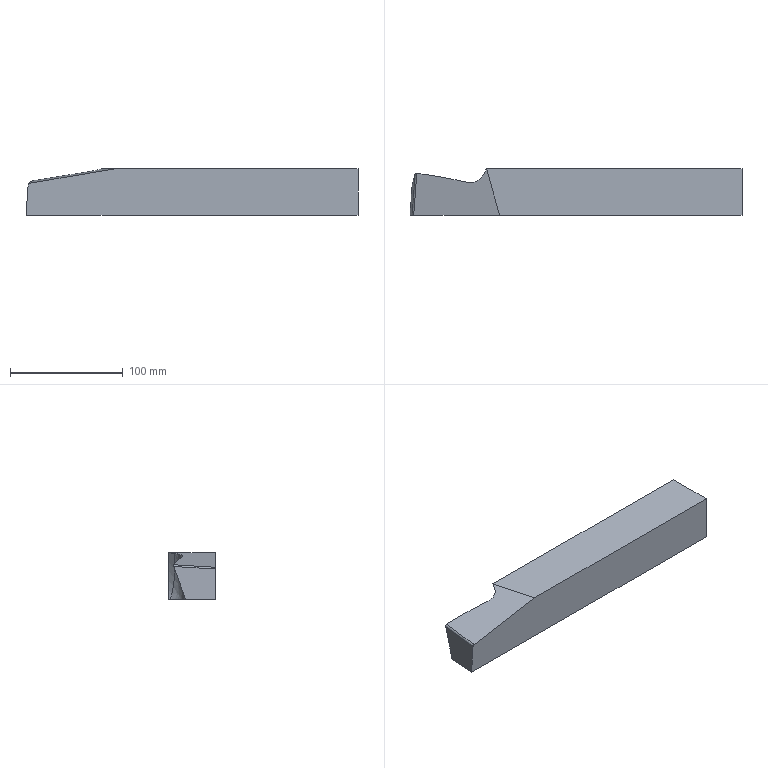Component | SolidWorks | LatheTool-1 | 1 solid | 11 faces | box 294.48 x 41.35 x 41.35 mm | volume 452255 mm3 | plane 7 | spline 3 | cylinder 1 | commonest cylinder face diameters 3.308 x1
STEP:
#1=COLOUR_RGB('',0.7922,0.8196,0.9333);
#2=FILL_AREA_STYLE_COLOUR('',#1);
#3=FILL_AREA_STYLE('',(#2));
#4=SURFACE_STYLE_FILL_AREA(#3);
#5=SURFACE_SIDE_STYLE('',(#4));
#6=SURFACE_STYLE_USAGE(.BOTH.,#5);
#7=PRESENTATION_STYLE_ASSIGNMENT((#6));
#8=CARTESIAN_POINT('',(-6.686,2.198,-3.286));
#9=VERTEX_POINT('',#8);
#10=CARTESIAN_POINT('',(-15.152,2.198,-3.286));
#11=VERTEX_POINT('',#10);
#12=CARTESIAN_POINT('',(-6.686,2.198,-3.286));
#13=DIRECTION('',(-1.,0.,0.));
#14=VECTOR('',#13,39.37);
#15=LINE('',#12,#14);
#16=EDGE_CURVE('',#9,#11,#15,.T.);
#17=ORIENTED_EDGE('',*,*,#16,.T.);
#18=CARTESIAN_POINT('',(-15.607,2.198,-1.658));
#19=VERTEX_POINT('',#18);
#20=CARTESIAN_POINT('',(-15.152,2.198,-3.286));
#21=CARTESIAN_POINT('',(-15.151,2.198,-3.214));
#22=CARTESIAN_POINT('',(-15.156,2.198,-3.143));
#23=CARTESIAN_POINT('',(-15.174,2.198,-3.003));
#24=CARTESIAN_POINT('',(-15.186,2.198,-2.934));
#25=CARTESIAN_POINT('',(-15.216,2.198,-2.796));
#26=CARTESIAN_POINT('',(-15.233,2.198,-2.728));
#27=CARTESIAN_POINT('',(-15.271,2.198,-2.591));
#28=CARTESIAN_POINT('',(-15.291,2.198,-2.523));
#29=CARTESIAN_POINT('',(-15.355,2.198,-2.321));
#30=CARTESIAN_POINT('',(-15.403,2.198,-2.187));
#31=CARTESIAN_POINT('',(-15.502,2.198,-1.921));
#32=CARTESIAN_POINT('',(-15.554,2.198,-1.789));
#33=CARTESIAN_POINT('',(-15.607,2.198,-1.658));
#34=B_SPLINE_CURVE_WITH_KNOTS('',3,(#20,#21,#22,#23,#24,#25,#26,#27,#28,#29,#30,#31,#32,#33),.UNSPECIFIED.,.F.,.F.,(4,2,2,2,2,2,4),(0.,0.00537,0.01074,0.01611,0.02148,0.03222,0.04296),.UNSPECIFIED.);
#35=EDGE_CURVE('',#11,#19,#34,.T.);
#36=ORIENTED_EDGE('',*,*,#35,.T.);
#37=CARTESIAN_POINT('',(-6.686,2.198,-1.658));
#38=VERTEX_POINT('',#37);
#39=CARTESIAN_POINT('',(-6.686,2.198,-1.658));
#40=DIRECTION('',(-1.,0.,0.));
#41=VECTOR('',#40,39.37);
#42=LINE('',#39,#41);
#43=EDGE_CURVE('',#38,#19,#42,.T.);
#44=ORIENTED_EDGE('',*,*,#43,.F.);
#45=CARTESIAN_POINT('',(-6.686,2.198,-1.658));
#46=DIRECTION('',(0.,0.,1.));
#47=VECTOR('',#46,39.37);
#48=LINE('',#45,#47);
#49=EDGE_CURVE('',#9,#38,#48,.T.);
#50=ORIENTED_EDGE('',*,*,#49,.F.);
#51=EDGE_LOOP('',(#17,#36,#44,#50));
#52=FACE_OUTER_BOUND('',#51,.T.);
#53=CARTESIAN_POINT('',(-6.686,2.198,-1.658));
#54=DIRECTION('',(0.,-1.,0.));
#55=DIRECTION('',(0.,0.,-1.));
#56=AXIS2_PLACEMENT_3D('',#53,#54,#55);
#57=PLANE('',#56);
#58=ADVANCED_FACE('',(#52),#57,.F.);
#59=CARTESIAN_POINT('',(-18.042,2.038,-2.079));
#60=VERTEX_POINT('',#59);
#61=CARTESIAN_POINT('',(-16.317,1.728,-1.801));
#62=VERTEX_POINT('',#61);
#63=CARTESIAN_POINT('',(-18.042,2.038,-2.079));
#64=CARTESIAN_POINT('',(-17.752,2.002,-2.031));
#65=CARTESIAN_POINT('',(-17.463,1.959,-1.984));
#66=CARTESIAN_POINT('',(-16.888,1.856,-1.892));
#67=CARTESIAN_POINT('',(-16.601,1.796,-1.846));
#68=CARTESIAN_POINT('',(-16.317,1.728,-1.801));
#69=B_SPLINE_CURVE_WITH_KNOTS('',3,(#63,#64,#65,#66,#67,#68),.UNSPECIFIED.,.F.,.F.,(4,2,4),(0.001307,0.02386,0.04641),.UNSPECIFIED.);
#70=EDGE_CURVE('',#60,#62,#69,.T.);
#71=ORIENTED_EDGE('',*,*,#70,.F.);
#72=CARTESIAN_POINT('',(-18.151,0.5701,-2.167));
#73=VERTEX_POINT('',#72);
#74=CARTESIAN_POINT('',(-18.151,0.5659,-2.167));
#75=DIRECTION('',(-0.07381,-0.9955,-0.05986));
#76=VECTOR('',#75,39.37);
#77=LINE('',#74,#76);
#78=EDGE_CURVE('',#60,#73,#77,.T.);
#79=ORIENTED_EDGE('',*,*,#78,.T.);
#80=CARTESIAN_POINT('',(-15.152,0.5701,-1.658));
#81=VERTEX_POINT('',#80);
#82=CARTESIAN_POINT('',(-6.923,0.5701,-0.2608));
#83=DIRECTION('',(-0.9859,0.,-0.1674));
#84=VECTOR('',#83,39.37);
#85=LINE('',#82,#84);
#86=EDGE_CURVE('',#81,#73,#85,.T.);
#87=ORIENTED_EDGE('',*,*,#86,.F.);
#88=CARTESIAN_POINT('',(-14.536,-1.628,-1.658));
#89=DIRECTION('',(0.2696,-0.963,0.));
#90=VECTOR('',#89,39.37);
#91=LINE('',#88,#90);
#92=EDGE_CURVE('',#19,#81,#91,.T.);
#93=ORIENTED_EDGE('',*,*,#92,.F.);
#94=CARTESIAN_POINT('',(-15.718,1.993,-1.686));
#95=VERTEX_POINT('',#94);
#96=CARTESIAN_POINT('',(-15.718,1.993,-1.686));
#97=CARTESIAN_POINT('',(-15.681,2.061,-1.677));
#98=CARTESIAN_POINT('',(-15.644,2.13,-1.667));
#99=CARTESIAN_POINT('',(-15.607,2.198,-1.658));
#100=B_SPLINE_CURVE_WITH_KNOTS('',3,(#96,#97,#98,#99),.UNSPECIFIED.,.F.,.F.,(4,4),(0.,0.005961),.UNSPECIFIED.);
#101=EDGE_CURVE('',#95,#19,#100,.T.);
#102=ORIENTED_EDGE('',*,*,#101,.F.);
#103=CARTESIAN_POINT('',(-15.718,1.993,-1.686));
#104=CARTESIAN_POINT('',(-15.732,1.966,-1.69));
#105=CARTESIAN_POINT('',(-15.748,1.942,-1.694));
#106=CARTESIAN_POINT('',(-15.783,1.895,-1.702));
#107=CARTESIAN_POINT('',(-15.803,1.874,-1.707));
#108=CARTESIAN_POINT('',(-15.847,1.833,-1.716));
#109=CARTESIAN_POINT('',(-15.87,1.815,-1.721));
#110=CARTESIAN_POINT('',(-15.919,1.784,-1.731));
#111=CARTESIAN_POINT('',(-15.945,1.77,-1.736));
#112=CARTESIAN_POINT('',(-15.999,1.746,-1.746));
#113=CARTESIAN_POINT('',(-16.027,1.737,-1.751));
#114=CARTESIAN_POINT('',(-16.083,1.722,-1.761));
#115=CARTESIAN_POINT('',(-16.112,1.718,-1.766));
#116=CARTESIAN_POINT('',(-16.156,1.714,-1.774));
#117=CARTESIAN_POINT('',(-16.171,1.713,-1.777));
#118=CARTESIAN_POINT('',(-16.2,1.713,-1.782));
#119=CARTESIAN_POINT('',(-16.215,1.714,-1.784));
#120=CARTESIAN_POINT('',(-16.259,1.717,-1.791));
#121=CARTESIAN_POINT('',(-16.288,1.721,-1.796));
#122=CARTESIAN_POINT('',(-16.317,1.728,-1.801));
#123=B_SPLINE_CURVE_WITH_KNOTS('',3,(#103,#104,#105,#106,#107,#108,#109,#110,#111,#112,#113,#114,#115,#116,#117,#118,#119,#120,#121,#122),.UNSPECIFIED.,.F.,.F.,(4,2,2,2,2,2,2,2,2,4),(0.,0.002256,0.004513,0.006769,0.009025,0.01128,0.01354,0.01467,0.01579,0.01805),.UNSPECIFIED.);
#124=EDGE_CURVE('',#95,#62,#123,.T.);
#125=ORIENTED_EDGE('',*,*,#124,.T.);
#126=EDGE_LOOP('',(#71,#79,#87,#93,#102,#125));
#127=FACE_OUTER_BOUND('',#126,.T.);
#128=CARTESIAN_POINT('',(-15.379,1.384,-1.658));
#129=DIRECTION('',(-0.1672,-0.04682,0.9848));
#130=DIRECTION('',(0.9859,0.,0.1674));
#131=AXIS2_PLACEMENT_3D('',#128,#129,#130);
#132=PLANE('',#131);
#133=ADVANCED_FACE('',(#127),#132,.T.);
#134=CARTESIAN_POINT('',(-18.28,0.5701,-3.286));
#135=VERTEX_POINT('',#134);
#136=CARTESIAN_POINT('',(-18.207,1.606,-3.286));
#137=VERTEX_POINT('',#136);
#138=CARTESIAN_POINT('',(-18.222,1.394,-3.286));
#139=DIRECTION('',(0.06976,0.9976,0.));
#140=VECTOR('',#139,39.37);
#141=LINE('',#138,#140);
#142=EDGE_CURVE('',#135,#137,#141,.T.);
#143=ORIENTED_EDGE('',*,*,#142,.T.);
#144=CARTESIAN_POINT('',(-15.7,1.606,-3.286));
#145=VERTEX_POINT('',#144);
#146=CARTESIAN_POINT('',(-15.152,1.606,-3.286));
#147=DIRECTION('',(-1.,0.,0.));
#148=VECTOR('',#147,39.37);
#149=LINE('',#146,#148);
#150=EDGE_CURVE('',#145,#137,#149,.T.);
#151=ORIENTED_EDGE('',*,*,#150,.F.);
#152=CARTESIAN_POINT('',(-15.152,2.153,-3.286));
#153=VERTEX_POINT('',#152);
#154=CARTESIAN_POINT('',(-15.7,1.606,-3.286));
#155=CARTESIAN_POINT('',(-15.663,1.606,-3.286));
#156=CARTESIAN_POINT('',(-15.628,1.609,-3.286));
#157=CARTESIAN_POINT('',(-15.575,1.619,-3.286));
#158=CARTESIAN_POINT('',(-15.558,1.624,-3.286));
#159=CARTESIAN_POINT('',(-15.524,1.634,-3.286));
#160=CARTESIAN_POINT('',(-15.506,1.64,-3.286));
#161=CARTESIAN_POINT('',(-15.457,1.661,-3.286));
#162=CARTESIAN_POINT('',(-15.425,1.678,-3.286));
#163=CARTESIAN_POINT('',(-15.381,1.707,-3.286));
#164=CARTESIAN_POINT('',(-15.366,1.718,-3.286));
#165=CARTESIAN_POINT('',(-15.338,1.741,-3.286));
#166=CARTESIAN_POINT('',(-15.325,1.753,-3.286));
#167=CARTESIAN_POINT('',(-15.287,1.791,-3.286));
#168=CARTESIAN_POINT('',(-15.264,1.818,-3.286));
#169=CARTESIAN_POINT('',(-15.234,1.863,-3.286));
#170=CARTESIAN_POINT('',(-15.225,1.879,-3.286));
#171=CARTESIAN_POINT('',(-15.208,1.91,-3.286));
#172=CARTESIAN_POINT('',(-15.193,1.943,-3.286));
#173=CARTESIAN_POINT('',(-15.181,1.976,-3.286));
#174=CARTESIAN_POINT('',(-15.17,2.011,-3.286));
#175=CARTESIAN_POINT('',(-15.166,2.028,-3.286));
#176=CARTESIAN_POINT('',(-15.155,2.081,-3.286));
#177=CARTESIAN_POINT('',(-15.152,2.117,-3.286));
#178=CARTESIAN_POINT('',(-15.152,2.153,-3.286));
#179=B_SPLINE_CURVE_WITH_KNOTS('',3,(#154,#155,#156,#157,#158,#159,#160,#161,#162,#163,#164,#165,#166,#167,#168,#169,#170,#171,#172,#173,#174,#175,#176,#177,#178),.UNSPECIFIED.,.F.,.F.,(4,2,2,2,2,2,2,2,2,1,2,2,4),(0.,0.002717,0.004076,0.005435,0.008152,0.009511,0.01087,0.01359,0.01495,0.0163,0.01766,0.01902,0.02174),.UNSPECIFIED.);
#180=EDGE_CURVE('',#145,#153,#179,.T.);
#181=ORIENTED_EDGE('',*,*,#180,.T.);
#182=CARTESIAN_POINT('',(-15.152,2.198,-3.286));
#183=DIRECTION('',(0.,-1.,0.));
#184=VECTOR('',#183,39.37);
#185=LINE('',#182,#184);
#186=EDGE_CURVE('',#11,#153,#185,.T.);
#187=ORIENTED_EDGE('',*,*,#186,.F.);
#188=ORIENTED_EDGE('',*,*,#16,.F.);
#189=CARTESIAN_POINT('',(-6.686,0.5701,-3.286));
#190=VERTEX_POINT('',#189);
#191=CARTESIAN_POINT('',(-6.686,0.5701,-3.286));
#192=DIRECTION('',(0.,1.,0.));
#193=VECTOR('',#192,39.37);
#194=LINE('',#191,#193);
#195=EDGE_CURVE('',#190,#9,#194,.T.);
#196=ORIENTED_EDGE('',*,*,#195,.F.);
#197=CARTESIAN_POINT('',(-6.686,0.5701,-3.286));
#198=DIRECTION('',(-1.,0.,0.));
#199=VECTOR('',#198,39.37);
#200=LINE('',#197,#199);
#201=EDGE_CURVE('',#190,#135,#200,.T.);
#202=ORIENTED_EDGE('',*,*,#201,.T.);
#203=EDGE_LOOP('',(#143,#151,#181,#187,#188,#196,#202));
#204=FACE_OUTER_BOUND('',#203,.T.);
#205=CARTESIAN_POINT('',(-6.686,0.5701,-3.286));
#206=DIRECTION('',(0.,0.,1.));
#207=DIRECTION('',(1.,0.,0.));
#208=AXIS2_PLACEMENT_3D('',#205,#206,#207);
#209=PLANE('',#208);
#210=ADVANCED_FACE('',(#204),#209,.F.);
#211=ORIENTED_EDGE('',*,*,#43,.T.);
#212=ORIENTED_EDGE('',*,*,#92,.T.);
#213=CARTESIAN_POINT('',(-6.686,0.5701,-1.658));
#214=VERTEX_POINT('',#213);
#215=CARTESIAN_POINT('',(-6.686,0.5701,-1.658));
#216=DIRECTION('',(-1.,0.,0.));
#217=VECTOR('',#216,39.37);
#218=LINE('',#215,#217);
#219=EDGE_CURVE('',#214,#81,#218,.T.);
#220=ORIENTED_EDGE('',*,*,#219,.F.);
#221=CARTESIAN_POINT('',(-6.686,0.5701,-1.658));
#222=DIRECTION('',(0.,-1.,0.));
#223=VECTOR('',#222,39.37);
#224=LINE('',#221,#223);
#225=EDGE_CURVE('',#38,#214,#224,.T.);
#226=ORIENTED_EDGE('',*,*,#225,.F.);
#227=EDGE_LOOP('',(#211,#212,#220,#226));
#228=FACE_OUTER_BOUND('',#227,.T.);
#229=CARTESIAN_POINT('',(-6.686,0.5701,-1.658));
#230=DIRECTION('',(0.,0.,-1.));
#231=DIRECTION('',(-1.,0.,0.));
#232=AXIS2_PLACEMENT_3D('',#229,#230,#231);
#233=PLANE('',#232);
#234=ADVANCED_FACE('',(#228),#233,.F.);
#235=ORIENTED_EDGE('',*,*,#86,.T.);
#236=CARTESIAN_POINT('',(-18.206,0.5701,-2.227));
#237=VERTEX_POINT('',#236);
#238=CARTESIAN_POINT('',(-18.151,0.5701,-2.167));
#239=CARTESIAN_POINT('',(-18.182,0.5701,-2.172));
#240=CARTESIAN_POINT('',(-18.203,0.5701,-2.196));
#241=CARTESIAN_POINT('',(-18.206,0.5701,-2.227));
#242=(BOUNDED_CURVE()B_SPLINE_CURVE(3,(#238,#239,#240,#241),.UNSPECIFIED.,.F.,.F.)B_SPLINE_CURVE_WITH_KNOTS((4,4),(4.197,5.534),.UNSPECIFIED.)CURVE()GEOMETRIC_REPRESENTATION_ITEM()RATIONAL_B_SPLINE_CURVE((1.,0.8565,0.8565,1.))REPRESENTATION_ITEM(''));
#243=EDGE_CURVE('',#73,#237,#242,.T.);
#244=ORIENTED_EDGE('',*,*,#243,.T.);
#245=CARTESIAN_POINT('',(-18.195,0.5701,-2.083));
#246=DIRECTION('',(-0.06993,0.,-0.9976));
#247=VECTOR('',#246,39.37);
#248=LINE('',#245,#247);
#249=EDGE_CURVE('',#237,#135,#248,.T.);
#250=ORIENTED_EDGE('',*,*,#249,.T.);
#251=ORIENTED_EDGE('',*,*,#201,.F.);
#252=CARTESIAN_POINT('',(-6.686,0.5701,-1.658));
#253=DIRECTION('',(0.,0.,-1.));
#254=VECTOR('',#253,39.37);
#255=LINE('',#252,#254);
#256=EDGE_CURVE('',#214,#190,#255,.T.);
#257=ORIENTED_EDGE('',*,*,#256,.F.);
#258=ORIENTED_EDGE('',*,*,#219,.T.);
#259=EDGE_LOOP('',(#235,#244,#250,#251,#257,#258));
#260=FACE_OUTER_BOUND('',#259,.T.);
#261=CARTESIAN_POINT('',(-6.686,0.5701,-1.658));
#262=DIRECTION('',(0.,1.,0.));
#263=DIRECTION('',(0.,0.,1.));
#264=AXIS2_PLACEMENT_3D('',#261,#262,#263);
#265=PLANE('',#264);
#266=ADVANCED_FACE('',(#260),#265,.F.);
#267=ORIENTED_EDGE('',*,*,#195,.T.);
#268=ORIENTED_EDGE('',*,*,#49,.T.);
#269=ORIENTED_EDGE('',*,*,#225,.T.);
#270=ORIENTED_EDGE('',*,*,#256,.T.);
#271=EDGE_LOOP('',(#267,#268,#269,#270));
#272=FACE_OUTER_BOUND('',#271,.T.);
#273=CARTESIAN_POINT('',(-6.686,1.384,-2.472));
#274=DIRECTION('',(-1.,0.,0.));
#275=DIRECTION('',(0.,0.,1.));
#276=AXIS2_PLACEMENT_3D('',#273,#274,#275);
#277=PLANE('',#276);
#278=ADVANCED_FACE('',(#272),#277,.F.);
#279=ORIENTED_EDGE('',*,*,#249,.F.);
#280=CARTESIAN_POINT('',(-18.098,2.025,-2.14));
#281=VERTEX_POINT('',#280);
#282=CARTESIAN_POINT('',(-18.096,2.047,-2.138));
#283=DIRECTION('',(0.07381,0.9955,0.05986));
#284=VECTOR('',#283,39.37);
#285=LINE('',#282,#284);
#286=EDGE_CURVE('',#237,#281,#285,.T.);
#287=ORIENTED_EDGE('',*,*,#286,.T.);
#288=CARTESIAN_POINT('',(-18.098,2.025,-2.14));
#289=CARTESIAN_POINT('',(-18.116,1.958,-2.332));
#290=CARTESIAN_POINT('',(-18.134,1.889,-2.523));
#291=CARTESIAN_POINT('',(-18.171,1.749,-2.905));
#292=CARTESIAN_POINT('',(-18.189,1.678,-3.096));
#293=CARTESIAN_POINT('',(-18.207,1.606,-3.286));
#294=B_SPLINE_CURVE_WITH_KNOTS('',3,(#288,#289,#290,#291,#292,#293),.UNSPECIFIED.,.F.,.F.,(4,2,4),(0.01977,0.03534,0.0509),.UNSPECIFIED.);
#295=EDGE_CURVE('',#281,#137,#294,.T.);
#296=ORIENTED_EDGE('',*,*,#295,.T.);
#297=ORIENTED_EDGE('',*,*,#142,.F.);
#298=EDGE_LOOP('',(#279,#287,#296,#297));
#299=FACE_OUTER_BOUND('',#298,.T.);
#300=CARTESIAN_POINT('',(-18.139,1.388,-2.087));
#301=DIRECTION('',(-0.9951,0.06959,0.06976));
#302=DIRECTION('',(0.06993,0.,0.9976));
#303=AXIS2_PLACEMENT_3D('',#300,#301,#302);
#304=PLANE('',#303);
#305=ADVANCED_FACE('',(#299),#304,.T.);
#306=ORIENTED_EDGE('',*,*,#186,.T.);
#307=CARTESIAN_POINT('',(-15.152,2.153,-3.286));
#308=CARTESIAN_POINT('',(-15.152,2.139,-3.253));
#309=CARTESIAN_POINT('',(-15.156,2.126,-3.219));
#310=CARTESIAN_POINT('',(-15.163,2.108,-3.169));
#311=CARTESIAN_POINT('',(-15.166,2.103,-3.152));
#312=CARTESIAN_POINT('',(-15.173,2.092,-3.118));
#313=CARTESIAN_POINT('',(-15.176,2.087,-3.101));
#314=CARTESIAN_POINT('',(-15.188,2.074,-3.05));
#315=CARTESIAN_POINT('',(-15.197,2.066,-3.016));
#316=CARTESIAN_POINT('',(-15.217,2.052,-2.949));
#317=CARTESIAN_POINT('',(-15.227,2.046,-2.915));
#318=CARTESIAN_POINT('',(-15.26,2.029,-2.814));
#319=CARTESIAN_POINT('',(-15.284,2.021,-2.748));
#320=CARTESIAN_POINT('',(-15.334,2.008,-2.614));
#321=CARTESIAN_POINT('',(-15.36,2.003,-2.547));
#322=CARTESIAN_POINT('',(-15.414,1.995,-2.414));
#323=CARTESIAN_POINT('',(-15.441,1.993,-2.348));
#324=CARTESIAN_POINT('',(-15.495,1.989,-2.215));
#325=CARTESIAN_POINT('',(-15.523,1.988,-2.149));
#326=CARTESIAN_POINT('',(-15.606,1.987,-1.951));
#327=CARTESIAN_POINT('',(-15.662,1.989,-1.819));
#328=CARTESIAN_POINT('',(-15.718,1.993,-1.686));
#329=B_SPLINE_CURVE_WITH_KNOTS('',3,(#307,#308,#309,#310,#311,#312,#313,#314,#315,#316,#317,#318,#319,#320,#321,#322,#323,#324,#325,#326,#327,#328),.UNSPECIFIED.,.F.,.F.,(4,2,2,2,2,2,2,2,2,2,4),(0.,0.002741,0.004112,0.005483,0.008224,0.01097,0.01645,0.02193,0.02741,0.0329,0.04386),.UNSPECIFIED.);
#330=EDGE_CURVE('',#153,#95,#329,.T.);
#331=ORIENTED_EDGE('',*,*,#330,.T.);
#332=ORIENTED_EDGE('',*,*,#101,.T.);
#333=ORIENTED_EDGE('',*,*,#35,.F.);
#334=EDGE_LOOP('',(#306,#331,#332,#333));
#335=FACE_OUTER_BOUND('',#334,.T.);
#336=CARTESIAN_POINT('',(-15.129,3.,-1.658));
#337=CARTESIAN_POINT('',(-15.136,2.733,-2.201));
#338=CARTESIAN_POINT('',(-15.144,2.465,-2.743));
#339=CARTESIAN_POINT('',(-15.152,2.198,-3.286));
#340=CARTESIAN_POINT('',(-15.197,2.886,-1.658));
#341=CARTESIAN_POINT('',(-15.182,2.64,-2.201));
#342=CARTESIAN_POINT('',(-15.167,2.394,-2.743));
#343=CARTESIAN_POINT('',(-15.152,2.149,-3.286));
#344=CARTESIAN_POINT('',(-15.334,2.657,-1.658));
#345=CARTESIAN_POINT('',(-15.273,2.454,-2.201));
#346=CARTESIAN_POINT('',(-15.212,2.252,-2.743));
#347=CARTESIAN_POINT('',(-15.152,2.05,-3.286));
#348=CARTESIAN_POINT('',(-15.539,2.313,-1.658));
#349=CARTESIAN_POINT('',(-15.41,2.176,-2.201));
#350=CARTESIAN_POINT('',(-15.281,2.039,-2.743));
#351=CARTESIAN_POINT('',(-15.152,1.902,-3.286));
#352=CARTESIAN_POINT('',(-15.744,1.97,-1.658));
#353=CARTESIAN_POINT('',(-15.546,1.898,-2.201));
#354=CARTESIAN_POINT('',(-15.349,1.826,-2.743));
#355=CARTESIAN_POINT('',(-15.152,1.754,-3.286));
#356=CARTESIAN_POINT('',(-15.88,1.741,-1.658));
#357=CARTESIAN_POINT('',(-15.637,1.712,-2.201));
#358=CARTESIAN_POINT('',(-15.395,1.684,-2.743));
#359=CARTESIAN_POINT('',(-15.152,1.655,-3.286));
#360=CARTESIAN_POINT('',(-15.949,1.627,-1.658));
#361=CARTESIAN_POINT('',(-15.683,1.62,-2.201));
#362=CARTESIAN_POINT('',(-15.417,1.613,-2.743));
#363=CARTESIAN_POINT('',(-15.152,1.606,-3.286));
#364=B_SPLINE_SURFACE_WITH_KNOTS('',3,3,((#336,#337,#338,#339),(#340,#341,#342,#343),(#344,#345,#346,#347),(#348,#349,#350,#351),(#352,#353,#354,#355),(#356,#357,#358,#359),(#360,#361,#362,#363)),.UNSPECIFIED.,.F.,.F.,.F.,(4,1,1,1,4),(4,4),(0.4983,0.5352,0.5722,0.6091,0.6461),(0.,1.),.UNSPECIFIED.);
#365=ADVANCED_FACE('',(#335),#364,.F.);
#366=ORIENTED_EDGE('',*,*,#295,.F.);
#367=CARTESIAN_POINT('',(-18.098,2.025,-2.14));
#368=CARTESIAN_POINT('',(-18.097,2.028,-2.133));
#369=CARTESIAN_POINT('',(-18.095,2.03,-2.126));
#370=CARTESIAN_POINT('',(-18.09,2.034,-2.112));
#371=CARTESIAN_POINT('',(-18.086,2.036,-2.106));
#372=CARTESIAN_POINT('',(-18.078,2.037,-2.098));
#373=CARTESIAN_POINT('',(-18.076,2.038,-2.095));
#374=CARTESIAN_POINT('',(-18.07,2.039,-2.09));
#375=CARTESIAN_POINT('',(-18.067,2.039,-2.088));
#376=CARTESIAN_POINT('',(-18.06,2.039,-2.085));
#377=CARTESIAN_POINT('',(-18.057,2.039,-2.083));
#378=CARTESIAN_POINT('',(-18.05,2.038,-2.081));
#379=CARTESIAN_POINT('',(-18.046,2.038,-2.08));
#380=CARTESIAN_POINT('',(-18.042,2.038,-2.079));
#381=B_SPLINE_CURVE_WITH_KNOTS('',3,(#367,#368,#369,#370,#371,#372,#373,#374,#375,#376,#377,#378,#379,#380),.UNSPECIFIED.,.F.,.F.,(4,2,2,2,2,2,4),(0.,0.0005692,0.001138,0.001423,0.001708,0.001992,0.002277),.UNSPECIFIED.);
#382=EDGE_CURVE('',#281,#60,#381,.T.);
#383=ORIENTED_EDGE('',*,*,#382,.T.);
#384=ORIENTED_EDGE('',*,*,#70,.T.);
#385=CARTESIAN_POINT('',(-16.317,1.728,-1.801));
#386=CARTESIAN_POINT('',(-16.256,1.715,-1.92));
#387=CARTESIAN_POINT('',(-16.195,1.703,-2.04));
#388=CARTESIAN_POINT('',(-16.077,1.681,-2.282));
#389=CARTESIAN_POINT('',(-16.019,1.671,-2.403));
#390=CARTESIAN_POINT('',(-15.935,1.656,-2.587));
#391=CARTESIAN_POINT('',(-15.907,1.652,-2.649));
#392=CARTESIAN_POINT('',(-15.854,1.643,-2.772));
#393=CARTESIAN_POINT('',(-15.829,1.638,-2.835));
#394=CARTESIAN_POINT('',(-15.793,1.631,-2.929));
#395=CARTESIAN_POINT('',(-15.781,1.629,-2.96));
#396=CARTESIAN_POINT('',(-15.759,1.625,-3.024));
#397=CARTESIAN_POINT('',(-15.748,1.622,-3.056));
#398=CARTESIAN_POINT('',(-15.729,1.618,-3.12));
#399=CARTESIAN_POINT('',(-15.72,1.616,-3.153));
#400=CARTESIAN_POINT('',(-15.709,1.612,-3.202));
#401=CARTESIAN_POINT('',(-15.705,1.611,-3.219));
#402=CARTESIAN_POINT('',(-15.702,1.609,-3.244));
#403=CARTESIAN_POINT('',(-15.701,1.608,-3.252));
#404=CARTESIAN_POINT('',(-15.7,1.607,-3.265));
#405=CARTESIAN_POINT('',(-15.699,1.607,-3.269));
#406=CARTESIAN_POINT('',(-15.699,1.606,-3.277));
#407=CARTESIAN_POINT('',(-15.699,1.606,-3.282));
#408=CARTESIAN_POINT('',(-15.7,1.606,-3.286));
#409=B_SPLINE_CURVE_WITH_KNOTS('',3,(#385,#386,#387,#388,#389,#390,#391,#392,#393,#394,#395,#396,#397,#398,#399,#400,#401,#402,#403,#404,#405,#406,#407,#408),.UNSPECIFIED.,.F.,.F.,(4,2,2,2,2,2,2,2,2,2,2,4),(0.004097,0.01438,0.02467,0.02981,0.03495,0.03753,0.0401,0.04267,0.04395,0.0446,0.04492,0.04524),.UNSPECIFIED.);
#410=EDGE_CURVE('',#62,#145,#409,.T.);
#411=ORIENTED_EDGE('',*,*,#410,.T.);
#412=ORIENTED_EDGE('',*,*,#150,.T.);
#413=EDGE_LOOP('',(#366,#383,#384,#411,#412));
#414=FACE_OUTER_BOUND('',#413,.T.);
#415=CARTESIAN_POINT('',(-15.949,1.627,-1.658));
#416=CARTESIAN_POINT('',(-15.683,1.62,-2.201));
#417=CARTESIAN_POINT('',(-15.417,1.613,-2.743));
#418=CARTESIAN_POINT('',(-15.152,1.606,-3.286));
#419=CARTESIAN_POINT('',(-16.126,1.674,-1.658));
#420=CARTESIAN_POINT('',(-15.883,1.651,-2.201));
#421=CARTESIAN_POINT('',(-15.639,1.628,-2.743));
#422=CARTESIAN_POINT('',(-15.396,1.606,-3.286));
#423=CARTESIAN_POINT('',(-16.482,1.769,-1.658));
#424=CARTESIAN_POINT('',(-16.283,1.715,-2.201));
#425=CARTESIAN_POINT('',(-16.083,1.66,-2.743));
#426=CARTESIAN_POINT('',(-15.884,1.606,-3.286));
#427=CARTESIAN_POINT('',(-17.015,1.912,-1.658));
#428=CARTESIAN_POINT('',(-16.882,1.81,-2.201));
#429=CARTESIAN_POINT('',(-16.75,1.708,-2.743));
#430=CARTESIAN_POINT('',(-16.617,1.606,-3.286));
#431=CARTESIAN_POINT('',(-17.549,2.055,-1.658));
#432=CARTESIAN_POINT('',(-17.482,1.905,-2.201));
#433=CARTESIAN_POINT('',(-17.416,1.755,-2.743));
#434=CARTESIAN_POINT('',(-17.349,1.606,-3.286));
#435=CARTESIAN_POINT('',(-17.904,2.15,-1.658));
#436=CARTESIAN_POINT('',(-17.882,1.969,-2.201));
#437=CARTESIAN_POINT('',(-17.86,1.787,-2.743));
#438=CARTESIAN_POINT('',(-17.838,1.606,-3.286));
#439=CARTESIAN_POINT('',(-18.082,2.198,-1.658));
#440=CARTESIAN_POINT('',(-18.082,2.001,-2.201));
#441=CARTESIAN_POINT('',(-18.082,1.803,-2.743));
#442=CARTESIAN_POINT('',(-18.082,1.606,-3.286));
#443=CARTESIAN_POINT('',(-18.092,2.201,-1.658));
#444=CARTESIAN_POINT('',(-18.093,2.002,-2.201));
#445=CARTESIAN_POINT('',(-18.094,1.804,-2.743));
#446=CARTESIAN_POINT('',(-18.096,1.606,-3.286));
#447=CARTESIAN_POINT('',(-18.102,2.203,-1.658));
#448=CARTESIAN_POINT('',(-18.105,2.004,-2.201));
#449=CARTESIAN_POINT('',(-18.107,1.805,-2.743));
#450=CARTESIAN_POINT('',(-18.11,1.606,-3.286));
#451=CARTESIAN_POINT('',(-18.112,2.206,-1.658));
#452=CARTESIAN_POINT('',(-18.116,2.006,-2.201));
#453=CARTESIAN_POINT('',(-18.12,1.806,-2.743));
#454=CARTESIAN_POINT('',(-18.123,1.606,-3.286));
#455=CARTESIAN_POINT('',(-18.132,2.212,-1.658));
#456=CARTESIAN_POINT('',(-18.139,2.01,-2.201));
#457=CARTESIAN_POINT('',(-18.145,1.808,-2.743));
#458=CARTESIAN_POINT('',(-18.151,1.606,-3.286));
#459=CARTESIAN_POINT('',(-18.153,2.217,-1.658));
#460=CARTESIAN_POINT('',(-18.162,2.013,-2.201));
#461=CARTESIAN_POINT('',(-18.171,1.809,-2.743));
#462=CARTESIAN_POINT('',(-18.179,1.606,-3.286));
#463=CARTESIAN_POINT('',(-18.173,2.223,-1.658));
#464=CARTESIAN_POINT('',(-18.185,2.017,-2.201));
#465=CARTESIAN_POINT('',(-18.196,1.811,-2.743));
#466=CARTESIAN_POINT('',(-18.207,1.606,-3.286));
#467=B_SPLINE_SURFACE_WITH_KNOTS('',3,3,((#415,#416,#417,#418),(#419,#420,#421,#422),(#423,#424,#425,#426),(#427,#428,#429,#430),(#431,#432,#433,#434),(#435,#436,#437,#438),(#439,#440,#441,#442),(#443,#444,#445,#446),(#447,#448,#449,#450),(#451,#452,#453,#454),(#455,#456,#457,#458),(#459,#460,#461,#462),(#463,#464,#465,#466)),.UNSPECIFIED.,.F.,.F.,.F.,(4,1,1,1,3,3,4),(4,4),(0.6461,0.7345,0.823,0.9115,1.,1.005,1.015),(0.,1.),.UNSPECIFIED.);
#468=ADVANCED_FACE('',(#414),#467,.F.);
#469=ORIENTED_EDGE('',*,*,#124,.F.);
#470=ORIENTED_EDGE('',*,*,#330,.F.);
#471=ORIENTED_EDGE('',*,*,#180,.F.);
#472=ORIENTED_EDGE('',*,*,#410,.F.);
#473=EDGE_LOOP('',(#469,#470,#471,#472));
#474=FACE_OUTER_BOUND('',#473,.T.);
#475=CARTESIAN_POINT('',(-15.164,2.219,-3.419));
#476=CARTESIAN_POINT('',(-15.08,1.598,-3.384));
#477=CARTESIAN_POINT('',(-15.7,1.606,-3.286));
#478=CARTESIAN_POINT('',(-15.163,2.215,-3.412));
#479=CARTESIAN_POINT('',(-15.083,1.598,-3.376));
#480=CARTESIAN_POINT('',(-15.7,1.606,-3.285));
#481=CARTESIAN_POINT('',(-15.162,2.212,-3.407));
#482=CARTESIAN_POINT('',(-15.086,1.599,-3.369));
#483=CARTESIAN_POINT('',(-15.7,1.606,-3.285));
#484=CARTESIAN_POINT('',(-15.16,2.207,-3.397));
#485=CARTESIAN_POINT('',(-15.091,1.6,-3.358));
#486=CARTESIAN_POINT('',(-15.699,1.606,-3.284));
#487=CARTESIAN_POINT('',(-15.159,2.205,-3.393));
#488=CARTESIAN_POINT('',(-15.094,1.6,-3.353));
#489=CARTESIAN_POINT('',(-15.699,1.606,-3.283));
#490=CARTESIAN_POINT('',(-15.157,2.199,-3.382));
#491=CARTESIAN_POINT('',(-15.1,1.601,-3.341));
#492=CARTESIAN_POINT('',(-15.699,1.606,-3.282));
#493=CARTESIAN_POINT('',(-15.156,2.196,-3.375));
#494=CARTESIAN_POINT('',(-15.104,1.601,-3.334));
#495=CARTESIAN_POINT('',(-15.699,1.606,-3.281));
#496=CARTESIAN_POINT('',(-15.155,2.19,-3.363));
#497=CARTESIAN_POINT('',(-15.11,1.602,-3.321));
#498=CARTESIAN_POINT('',(-15.699,1.606,-3.279));
#499=CARTESIAN_POINT('',(-15.154,2.187,-3.358));
#500=CARTESIAN_POINT('',(-15.113,1.603,-3.316));
#501=CARTESIAN_POINT('',(-15.699,1.606,-3.278));
#502=CARTESIAN_POINT('',(-15.153,2.182,-3.349));
#503=CARTESIAN_POINT('',(-15.118,1.603,-3.305));
#504=CARTESIAN_POINT('',(-15.699,1.606,-3.276));
#505=CARTESIAN_POINT('',(-15.153,2.18,-3.344));
#506=CARTESIAN_POINT('',(-15.121,1.604,-3.301));
#507=CARTESIAN_POINT('',(-15.699,1.606,-3.275));
#508=CARTESIAN_POINT('',(-15.152,2.174,-3.331));
#509=CARTESIAN_POINT('',(-15.128,1.604,-3.288));
#510=CARTESIAN_POINT('',(-15.699,1.607,-3.272));
#511=CARTESIAN_POINT('',(-15.152,2.17,-3.324));
#512=CARTESIAN_POINT('',(-15.132,1.605,-3.281));
#513=CARTESIAN_POINT('',(-15.699,1.607,-3.27));
#514=CARTESIAN_POINT('',(-15.151,2.164,-3.31));
#515=CARTESIAN_POINT('',(-15.14,1.606,-3.267));
#516=CARTESIAN_POINT('',(-15.7,1.607,-3.266));
#517=CARTESIAN_POINT('',(-15.151,2.161,-3.303));
#518=CARTESIAN_POINT('',(-15.143,1.606,-3.261));
#519=CARTESIAN_POINT('',(-15.7,1.607,-3.264));
#520=CARTESIAN_POINT('',(-15.151,2.153,-3.285));
#521=CARTESIAN_POINT('',(-15.153,1.607,-3.244));
#522=CARTESIAN_POINT('',(-15.7,1.608,-3.257));
#523=CARTESIAN_POINT('',(-15.152,2.148,-3.274));
#524=CARTESIAN_POINT('',(-15.159,1.607,-3.234));
#525=CARTESIAN_POINT('',(-15.701,1.608,-3.253));
#526=CARTESIAN_POINT('',(-15.153,2.14,-3.254));
#527=CARTESIAN_POINT('',(-15.169,1.608,-3.215));
#528=CARTESIAN_POINT('',(-15.702,1.609,-3.245));
#529=CARTESIAN_POINT('',(-15.154,2.136,-3.245));
#530=CARTESIAN_POINT('',(-15.174,1.609,-3.207));
#531=CARTESIAN_POINT('',(-15.702,1.609,-3.241));
#532=CARTESIAN_POINT('',(-15.156,2.126,-3.218));
#533=CARTESIAN_POINT('',(-15.188,1.61,-3.183));
#534=CARTESIAN_POINT('',(-15.704,1.61,-3.229));
#535=CARTESIAN_POINT('',(-15.158,2.12,-3.202));
#536=CARTESIAN_POINT('',(-15.196,1.61,-3.169));
#537=CARTESIAN_POINT('',(-15.705,1.611,-3.221));
#538=CARTESIAN_POINT('',(-15.163,2.109,-3.172));
#539=CARTESIAN_POINT('',(-15.211,1.611,-3.142));
#540=CARTESIAN_POINT('',(-15.708,1.612,-3.205));
#541=CARTESIAN_POINT('',(-15.165,2.105,-3.158));
#542=CARTESIAN_POINT('',(-15.218,1.612,-3.13));
#543=CARTESIAN_POINT('',(-15.71,1.612,-3.197));
#544=CARTESIAN_POINT('',(-15.173,2.092,-3.118));
#545=CARTESIAN_POINT('',(-15.237,1.613,-3.094));
#546=CARTESIAN_POINT('',(-15.715,1.614,-3.173));
#547=CARTESIAN_POINT('',(-15.178,2.085,-3.094));
#548=CARTESIAN_POINT('',(-15.249,1.613,-3.073));
#549=CARTESIAN_POINT('',(-15.719,1.615,-3.156));
#550=CARTESIAN_POINT('',(-15.189,2.073,-3.047));
#551=CARTESIAN_POINT('',(-15.271,1.615,-3.031));
#552=CARTESIAN_POINT('',(-15.728,1.618,-3.124));
#553=CARTESIAN_POINT('',(-15.195,2.068,-3.025));
#554=CARTESIAN_POINT('',(-15.281,1.615,-3.012));
#555=CARTESIAN_POINT('',(-15.732,1.619,-3.108));
#556=CARTESIAN_POINT('',(-15.213,2.054,-2.961));
#557=CARTESIAN_POINT('',(-15.311,1.616,-2.955));
#558=CARTESIAN_POINT('',(-15.747,1.622,-3.06));
#559=CARTESIAN_POINT('',(-15.225,2.047,-2.921));
#560=CARTESIAN_POINT('',(-15.329,1.617,-2.919));
#561=CARTESIAN_POINT('',(-15.757,1.624,-3.029));
#562=CARTESIAN_POINT('',(-15.25,2.034,-2.845));
#563=CARTESIAN_POINT('',(-15.364,1.619,-2.849));
#564=CARTESIAN_POINT('',(-15.779,1.629,-2.965));
#565=CARTESIAN_POINT('',(-15.263,2.029,-2.808));
#566=CARTESIAN_POINT('',(-15.381,1.619,-2.815));
#567=CARTESIAN_POINT('',(-15.791,1.631,-2.934));
#568=CARTESIAN_POINT('',(-15.289,2.02,-2.735));
#569=CARTESIAN_POINT('',(-15.415,1.62,-2.747));
#570=CARTESIAN_POINT('',(-15.815,1.635,-2.871));
#571=CARTESIAN_POINT('',(-15.302,2.016,-2.7));
#572=CARTESIAN_POINT('',(-15.431,1.621,-2.714));
#573=CARTESIAN_POINT('',(-15.827,1.638,-2.84));
#574=CARTESIAN_POINT('',(-15.328,2.01,-2.63));
#575=CARTESIAN_POINT('',(-15.463,1.622,-2.649));
#576=CARTESIAN_POINT('',(-15.853,1.642,-2.777));
#577=CARTESIAN_POINT('',(-15.342,2.007,-2.596));
#578=CARTESIAN_POINT('',(-15.479,1.623,-2.616));
#579=CARTESIAN_POINT('',(-15.866,1.644,-2.746));
#580=CARTESIAN_POINT('',(-15.381,1.999,-2.494));
#581=CARTESIAN_POINT('',(-15.526,1.624,-2.52));
#582=CARTESIAN_POINT('',(-15.906,1.651,-2.653));
#583=CARTESIAN_POINT('',(-15.408,1.996,-2.428));
#584=CARTESIAN_POINT('',(-15.557,1.625,-2.456));
#585=CARTESIAN_POINT('',(-15.933,1.656,-2.591));
#586=CARTESIAN_POINT('',(-15.462,1.991,-2.296));
#587=CARTESIAN_POINT('',(-15.619,1.627,-2.329));
#588=CARTESIAN_POINT('',(-15.99,1.666,-2.467));
#589=CARTESIAN_POINT('',(-15.489,1.989,-2.231));
#590=CARTESIAN_POINT('',(-15.65,1.629,-2.266));
#591=CARTESIAN_POINT('',(-16.018,1.671,-2.405));
#592=CARTESIAN_POINT('',(-15.542,1.988,-2.102));
#593=CARTESIAN_POINT('',(-15.71,1.631,-2.14));
#594=CARTESIAN_POINT('',(-16.077,1.681,-2.282));
#595=CARTESIAN_POINT('',(-15.569,1.988,-2.038));
#596=CARTESIAN_POINT('',(-15.741,1.632,-2.077));
#597=CARTESIAN_POINT('',(-16.107,1.687,-2.221));
#598=CARTESIAN_POINT('',(-15.65,1.989,-1.846));
#599=CARTESIAN_POINT('',(-15.832,1.635,-1.889));
#600=CARTESIAN_POINT('',(-16.197,1.703,-2.037));
#601=CARTESIAN_POINT('',(-15.704,1.991,-1.719));
#602=CARTESIAN_POINT('',(-15.892,1.637,-1.764));
#603=CARTESIAN_POINT('',(-16.259,1.716,-1.914));
#604=CARTESIAN_POINT('',(-15.757,1.996,-1.593));
#605=CARTESIAN_POINT('',(-15.952,1.64,-1.64));
#606=CARTESIAN_POINT('',(-16.321,1.729,-1.792));
#607=(BOUNDED_SURFACE()B_SPLINE_SURFACE(3,2,((#475,#476,#477),(#478,#479,#480),(#481,#482,#483),(#484,#485,#486),(#487,#488,#489),(#490,#491,#492),(#493,#494,#495),(#496,#497,#498),(#499,#500,#501),(#502,#503,#504),(#505,#506,#507),(#508,#509,#510),(#511,#512,#513),(#514,#515,#516),(#517,#518,#519),(#520,#521,#522),(#523,#524,#525),(#526,#527,#528),(#529,#530,#531),(#532,#533,#534),(#535,#536,#537),(#538,#539,#540),(#541,#542,#543),(#544,#545,#546),(#547,#548,#549),(#550,#551,#552),(#553,#554,#555),(#556,#557,#558),(#559,#560,#561),(#562,#563,#564),(#565,#566,#567),(#568,#569,#570),(#571,#572,#573),(#574,#575,#576),(#577,#578,#579),(#580,#581,#582),(#583,#584,#585),(#586,#587,#588),(#589,#590,#591),(#592,#593,#594),(#595,#596,#597),(#598,#599,#600),(#601,#602,#603),(#604,#605,#606)),.UNSPECIFIED.,.F.,.F.,.F.)B_SPLINE_SURFACE_WITH_KNOTS((4,2,2,2,2,2,2,2,2,2,2,2,2,2,2,2,2,2,2,2,2,4),(3,3),(-0.0001349,-0.00009452,-0.00005409,0.00002676,0.0001076,0.0001885,0.0003502,0.0005119,0.0008353,0.001159,0.001805,0.002452,0.003746,0.00504,0.007627,0.01021,0.0128,0.01539,0.02056,0.02574,0.03091,0.04126),(0.,1.),.UNSPECIFIED.)GEOMETRIC_REPRESENTATION_ITEM()RATIONAL_B_SPLINE_SURFACE(((1.,0.657,1.),(1.,0.6599,1.),(1.,0.6621,1.),(1.,0.666,1.),(1.,0.6677,1.),(1.,0.6724,1.),(1.,0.6749,1.),(1.,0.6795,1.),(1.,0.6815,1.),(1.,0.6851,1.),(1.,0.6867,1.),(1.,0.6914,1.),(1.,0.694,1.),(1.,0.6988,1.),(1.,0.7009,1.),(1.,0.7069,1.),(1.,0.7102,1.),(1.,0.7162,1.),(1.,0.7188,1.),(1.,0.7261,1.),(1.,0.7301,1.),(1.,0.7372,1.),(1.,0.7403,1.),(1.,0.7487,1.),(1.,0.7533,1.),(1.,0.7611,1.),(1.,0.7644,1.),(1.,0.7733,1.),(1.,0.7779,1.),(1.,0.7855,1.),(1.,0.7885,1.),(1.,0.7938,1.),(1.,0.796,1.),(1.,0.7997,1.),(1.,0.8012,1.),(1.,0.8051,1.),(1.,0.8068,1.),(1.,0.809,1.),(1.,0.8096,1.),(1.,0.8098,1.),(1.,0.8094,1.),(1.,0.8074,1.),(1.,0.8047,1.),(1.,0.8009,1.)))REPRESENTATION_ITEM('')SURFACE());
#608=ADVANCED_FACE('',(#474),#607,.F.);
#609=ORIENTED_EDGE('',*,*,#382,.F.);
#610=ORIENTED_EDGE('',*,*,#286,.F.);
#611=ORIENTED_EDGE('',*,*,#243,.F.);
#612=ORIENTED_EDGE('',*,*,#78,.F.);
#613=EDGE_LOOP('',(#609,#610,#611,#612));
#614=FACE_OUTER_BOUND('',#613,.T.);
#615=CARTESIAN_POINT('',(-18.063,1.614,-2.169));
#616=DIRECTION('',(-0.07381,-0.9955,-0.05986));
#617=DIRECTION('',(0.9973,-0.07394,0.));
#618=AXIS2_PLACEMENT_3D('',#615,#616,#617);
#619=CYLINDRICAL_SURFACE('',#618,0.06512);
#620=ADVANCED_FACE('',(#614),#619,.T.);
#621=CLOSED_SHELL('',(#58,#133,#210,#234,#266,#278,#305,#365,#468,#608,#620));
#622=MANIFOLD_SOLID_BREP('',#621);
#623=STYLED_ITEM('',(#7),#622);
#624=(LENGTH_UNIT()NAMED_UNIT(*)SI_UNIT($,.METRE.));
#625=LENGTH_MEASURE_WITH_UNIT(LENGTH_MEASURE(0.0254),#624);
#626=DIMENSIONAL_EXPONENTS(1.,0.,0.,0.,0.,0.,0.);
#627=(CONVERSION_BASED_UNIT('',#625)LENGTH_UNIT()NAMED_UNIT(#626));
#628=UNCERTAINTY_MEASURE_WITH_UNIT(LENGTH_MEASURE(0.00001),#627,'','');
#629=(NAMED_UNIT(*)PLANE_ANGLE_UNIT()SI_UNIT($,.RADIAN.));
#630=(NAMED_UNIT(*)SI_UNIT($,.STERADIAN.)SOLID_ANGLE_UNIT());
#631=(GEOMETRIC_REPRESENTATION_CONTEXT(3)GLOBAL_UNCERTAINTY_ASSIGNED_CONTEXT((#628))GLOBAL_UNIT_ASSIGNED_CONTEXT((#627,#629,#630))REPRESENTATION_CONTEXT('',''));
#632=MECHANICAL_DESIGN_GEOMETRIC_PRESENTATION_REPRESENTATION('',(#623),#631);
#633=CARTESIAN_POINT('',(0.,0.,0.));
#634=DIRECTION('',(0.,0.,1.));
#635=DIRECTION('',(1.,0.,0.));
#636=AXIS2_PLACEMENT_3D('',#633,#634,#635);
#637=(LENGTH_UNIT()NAMED_UNIT(*)SI_UNIT($,.METRE.));
#638=LENGTH_MEASURE_WITH_UNIT(LENGTH_MEASURE(0.0254),#637);
#639=DIMENSIONAL_EXPONENTS(1.,0.,0.,0.,0.,0.,0.);
#640=(CONVERSION_BASED_UNIT('',#638)LENGTH_UNIT()NAMED_UNIT(#639));
#641=UNCERTAINTY_MEASURE_WITH_UNIT(LENGTH_MEASURE(0.00001),#640,'','');
#642=(NAMED_UNIT(*)PLANE_ANGLE_UNIT()SI_UNIT($,.RADIAN.));
#643=(NAMED_UNIT(*)SI_UNIT($,.STERADIAN.)SOLID_ANGLE_UNIT());
#644=(GEOMETRIC_REPRESENTATION_CONTEXT(3)GLOBAL_UNCERTAINTY_ASSIGNED_CONTEXT((#641))GLOBAL_UNIT_ASSIGNED_CONTEXT((#640,#642,#643))REPRESENTATION_CONTEXT('',''));
#645=ADVANCED_BREP_SHAPE_REPRESENTATION('',(#622,#636),#644);
#646=PRESENTATION_LAYER_ASSIGNMENT('','',(#623));